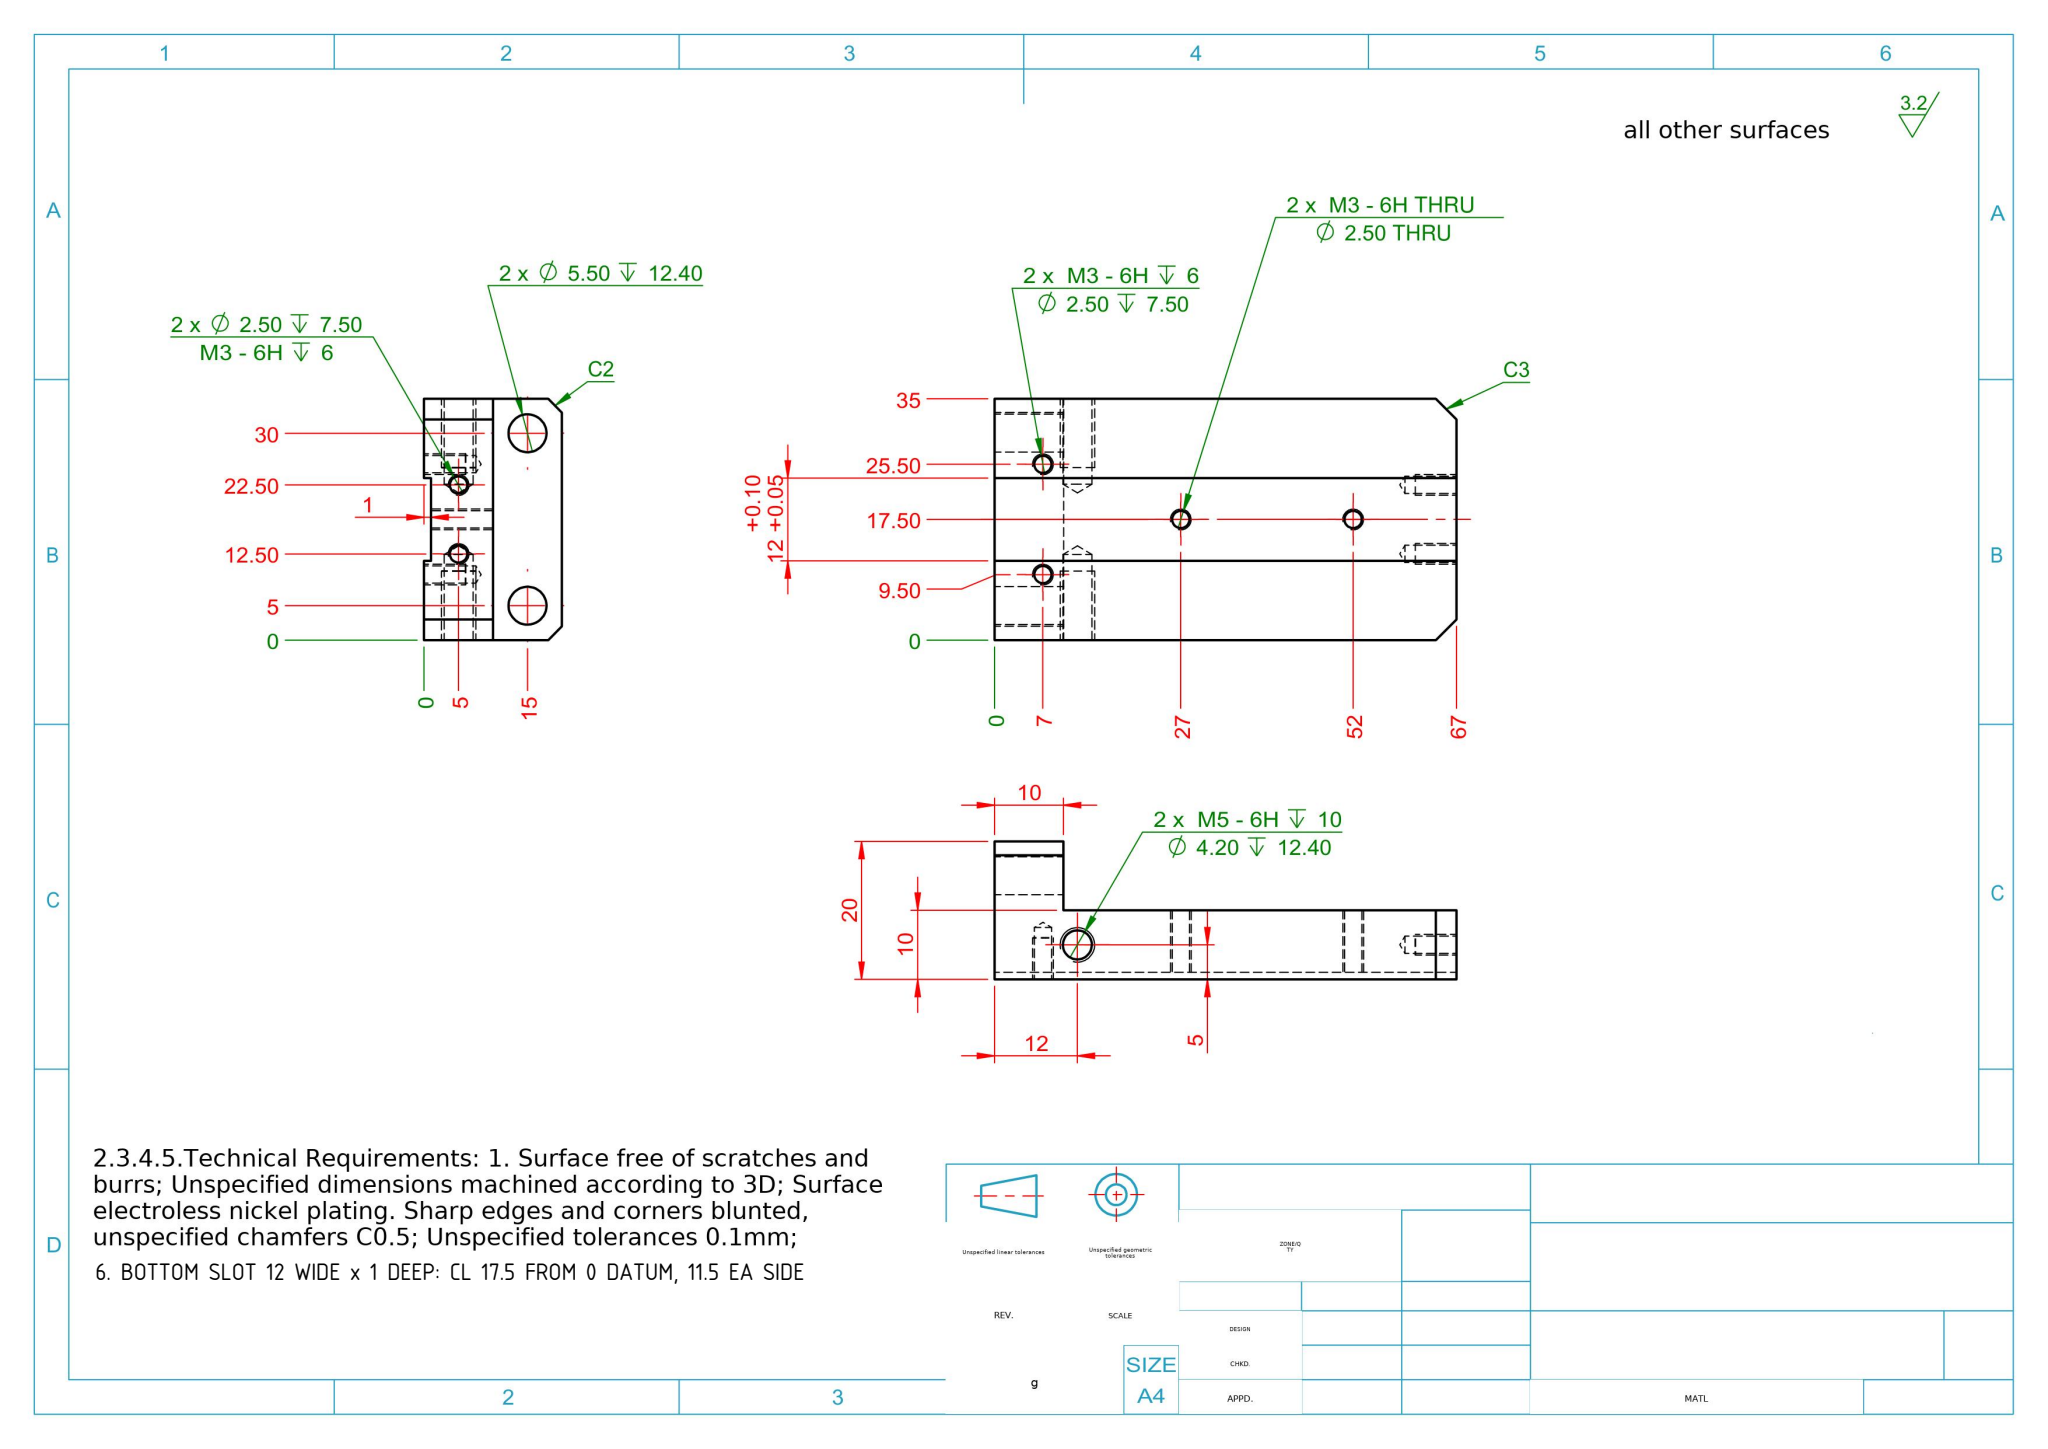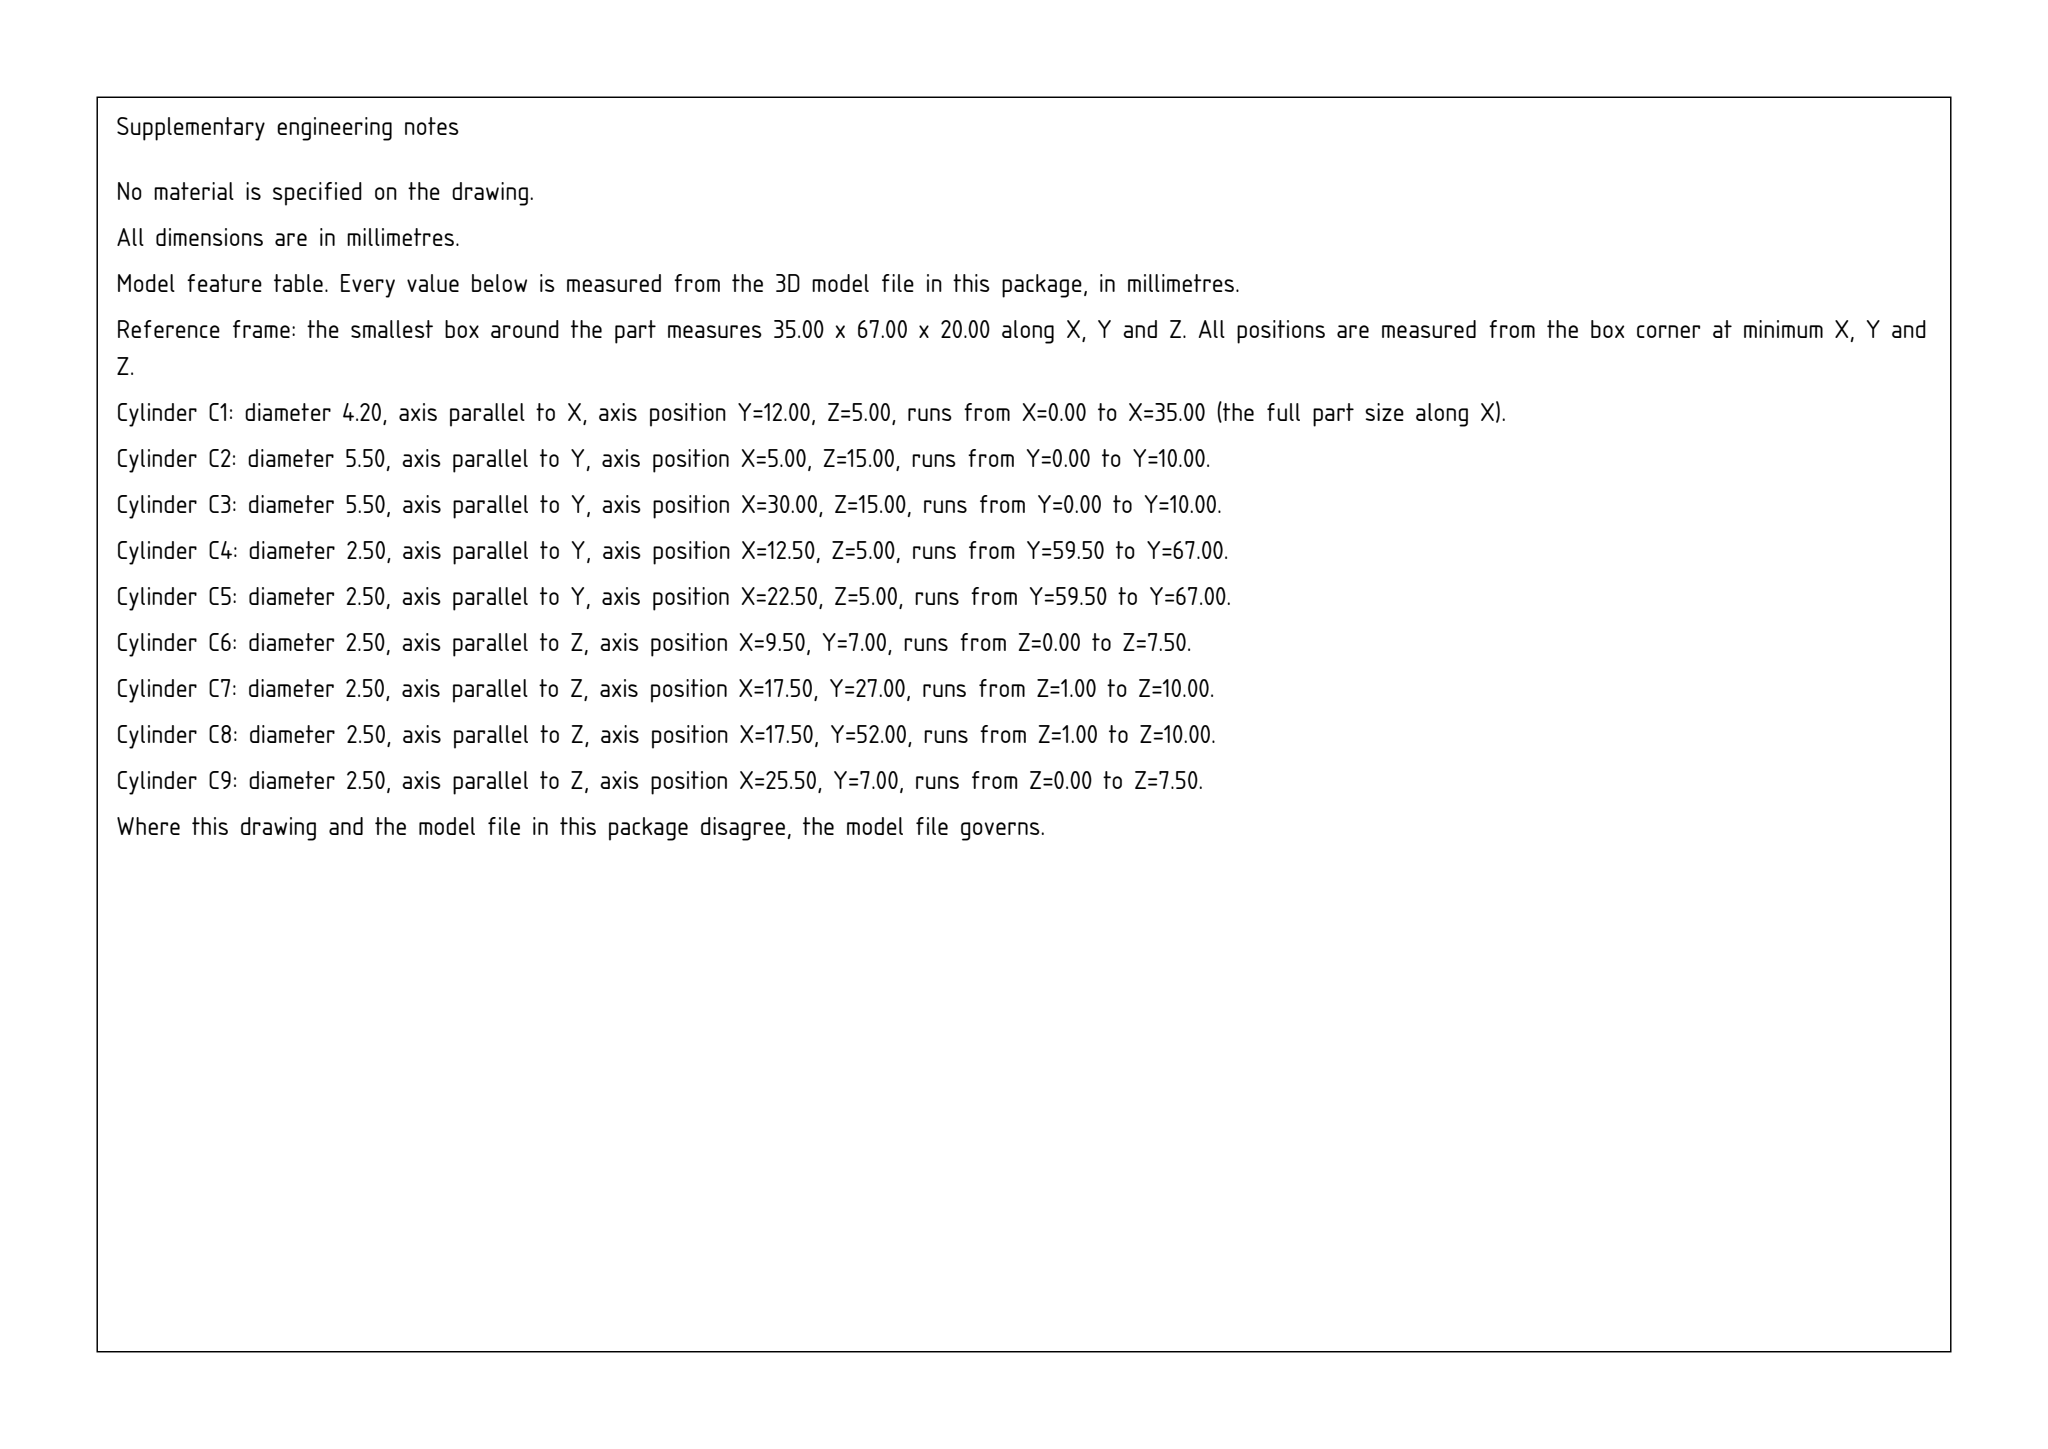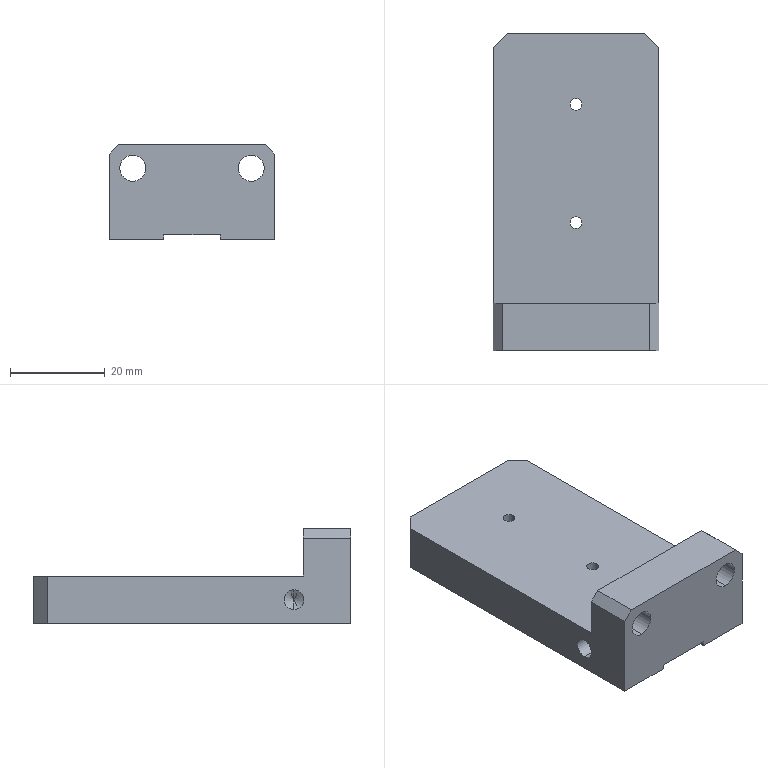Part | SolidWorks | mm | material S45C | 1 solid | 48 faces | box 35 x 67 x 20 mm | volume 24945 mm3 | cylinder 20 | plane 16 | cone 12 | commonest cylinder face diameters 2.5 x12 5.5 x4 4.2 x4
Drawing notes:
BOTTOM SLOT 12 WIDE x 1 DEEP: CL 17.5 FROM 0 DATUM, 11.5 EA SIDE | from the solid: Planes x=11.5 and x=23.5 (extent z 0-1, y 0-67) with floor z=1.0 between them; bbox X=35, so slot CL at x=17.5, 11.5 from each side face (x=0, x=35)
build123d program:
from build123d import *

# Parameters (mm, degrees)
SKETCH1_W                = 35
SKETCH1_H                = 67
BOSS_EXTRUDE1_DEPTH      = 10
SKETCH4_W                = 12
SKETCH4_H                = 67
CUT_EXTRUDE1_DEPTH       = 1
M3_TAPPED_HOLE1_D        = 2.5
M3_TAPPED_HOLE1_DEPTH    = 7.5
M3_TAPPED_HOLE1_TIP      = 0.7511
CHAMFER1_SIZE            = 3
SKETCH11_W               = 35
SKETCH11_H               = 10
BOSS_EXTRUDE2_DEPTH      = 10
M3_TAPPED_HOLE2_D        = 2.5
M3_TAPPED_HOLE2_DEPTH    = 7.5
M3_TAPPED_HOLE2_TIP      = 0.7511
M5_CLEARANCE_HOLE1_D     = 5.5
M5_CLEARANCE_HOLE1_DEPTH = 12.4
M5_CLEARANCE_HOLE1_TIP   = 1.652
CHAMFER2_SIZE            = 2
M3_TAPPED_HOLE3_D        = 2.5


with BuildPart() as part:
    # Sketch1 → Boss-Extrude1 (new body)
    with BuildSketch(Plane.XY):
        Rectangle(SKETCH1_W, SKETCH1_H)
    extrude(amount=BOSS_EXTRUDE1_DEPTH)

    # Sketch3 → M5 Tapped Hole1 (revolve, cut)
    with BuildSketch(Plane(origin=(17.5, -21.5, 5), x_dir=(0, 0, -1), z_dir=(0, 1, 0))):
        Polygon((0, 0), (0, 13.662), (2.1, 12.4), (2.1, 0), align=None)
    m5_tapped_hole1 = revolve(axis=Axis((23.85, -21.5, 5), (-1, 0, 0)), mode=Mode.SUBTRACT)

    # Sketch4 → Cut-Extrude1 (cut)
    with BuildSketch(Plane(origin=(0, 0, 0), x_dir=(-1, 0, 0), z_dir=(0, 0, -1))):
        Rectangle(SKETCH4_W, SKETCH4_H)
    extrude(amount=-CUT_EXTRUDE1_DEPTH, mode=Mode.SUBTRACT)

    # M3 Tapped Hole1
    with Locations(Plane(origin=(0, 33.5, 0), x_dir=(1, 0, 0), z_dir=(0, 1, 0))):
        with Locations((5, -5), (-5, -5)):
            Hole(M3_TAPPED_HOLE1_D / 2, depth=M3_TAPPED_HOLE1_DEPTH)
            with Locations((0, 0, -(M3_TAPPED_HOLE1_DEPTH + M3_TAPPED_HOLE1_TIP / 2))):  # 118° drill point
                Cone(0, M3_TAPPED_HOLE1_D / 2, M3_TAPPED_HOLE1_TIP, mode=Mode.SUBTRACT)

    # Chamfer1
    chamfer1_edges = [part.edges().sort_by_distance(p)[0] for p in [
        (-17.5, 33.5, 5),
        (17.5, 33.5, 5),
    ]]
    chamfer(chamfer1_edges, length=CHAMFER1_SIZE)

    # Mirror1: M5 Tapped Hole1 across plane
    add(m5_tapped_hole1.mirror(Plane(origin=(0, 0, 0), x_dir=(0, 0, 1), z_dir=(1, 0, 0))), mode=Mode.SUBTRACT)

    # Sketch11 → Boss-Extrude2 (add)
    with BuildSketch(Plane.XY.offset(10)):
        with Locations((0, -28.5)):
            Rectangle(SKETCH11_W, SKETCH11_H)
    extrude(amount=BOSS_EXTRUDE2_DEPTH)

    # M3 Tapped Hole2
    with Locations(Plane(origin=(0, 0, 0), x_dir=(-1, 0, 0), z_dir=(0, 0, -1))):
        with Locations((-8, -26.5), (8, -26.5)):
            Hole(M3_TAPPED_HOLE2_D / 2, depth=M3_TAPPED_HOLE2_DEPTH)
            with Locations((0, 0, -(M3_TAPPED_HOLE2_DEPTH + M3_TAPPED_HOLE2_TIP / 2))):  # 118° drill point
                Cone(0, M3_TAPPED_HOLE2_D / 2, M3_TAPPED_HOLE2_TIP, mode=Mode.SUBTRACT)

    # M5 Clearance Hole1
    with Locations(Plane(origin=(0, -23.5, 0), x_dir=(1, 0, 0), z_dir=(0, 1, 0))):
        with Locations((-12.5, -15), (12.5, -15)):
            Hole(M5_CLEARANCE_HOLE1_D / 2, depth=M5_CLEARANCE_HOLE1_DEPTH)
            with Locations((0, 0, -(M5_CLEARANCE_HOLE1_DEPTH + M5_CLEARANCE_HOLE1_TIP / 2))):  # 118° drill point
                Cone(0, M5_CLEARANCE_HOLE1_D / 2, M5_CLEARANCE_HOLE1_TIP, mode=Mode.SUBTRACT)

    # Chamfer2
    chamfer2_edges = [part.edges().sort_by_distance(p)[0] for p in [
        (-17.5, -28.5, 20),
        (17.5, -28.5, 20),
    ]]
    chamfer(chamfer2_edges, length=CHAMFER2_SIZE)

    # M3 Tapped Hole3 (through all)
    with Locations(Plane(origin=(0, 0, 1), x_dir=(-1, 0, 0), z_dir=(0, 0, -1))):
        with Locations((0, 18.5), (0, -6.5)):
            Hole(M3_TAPPED_HOLE3_D / 2)


solid = part.part